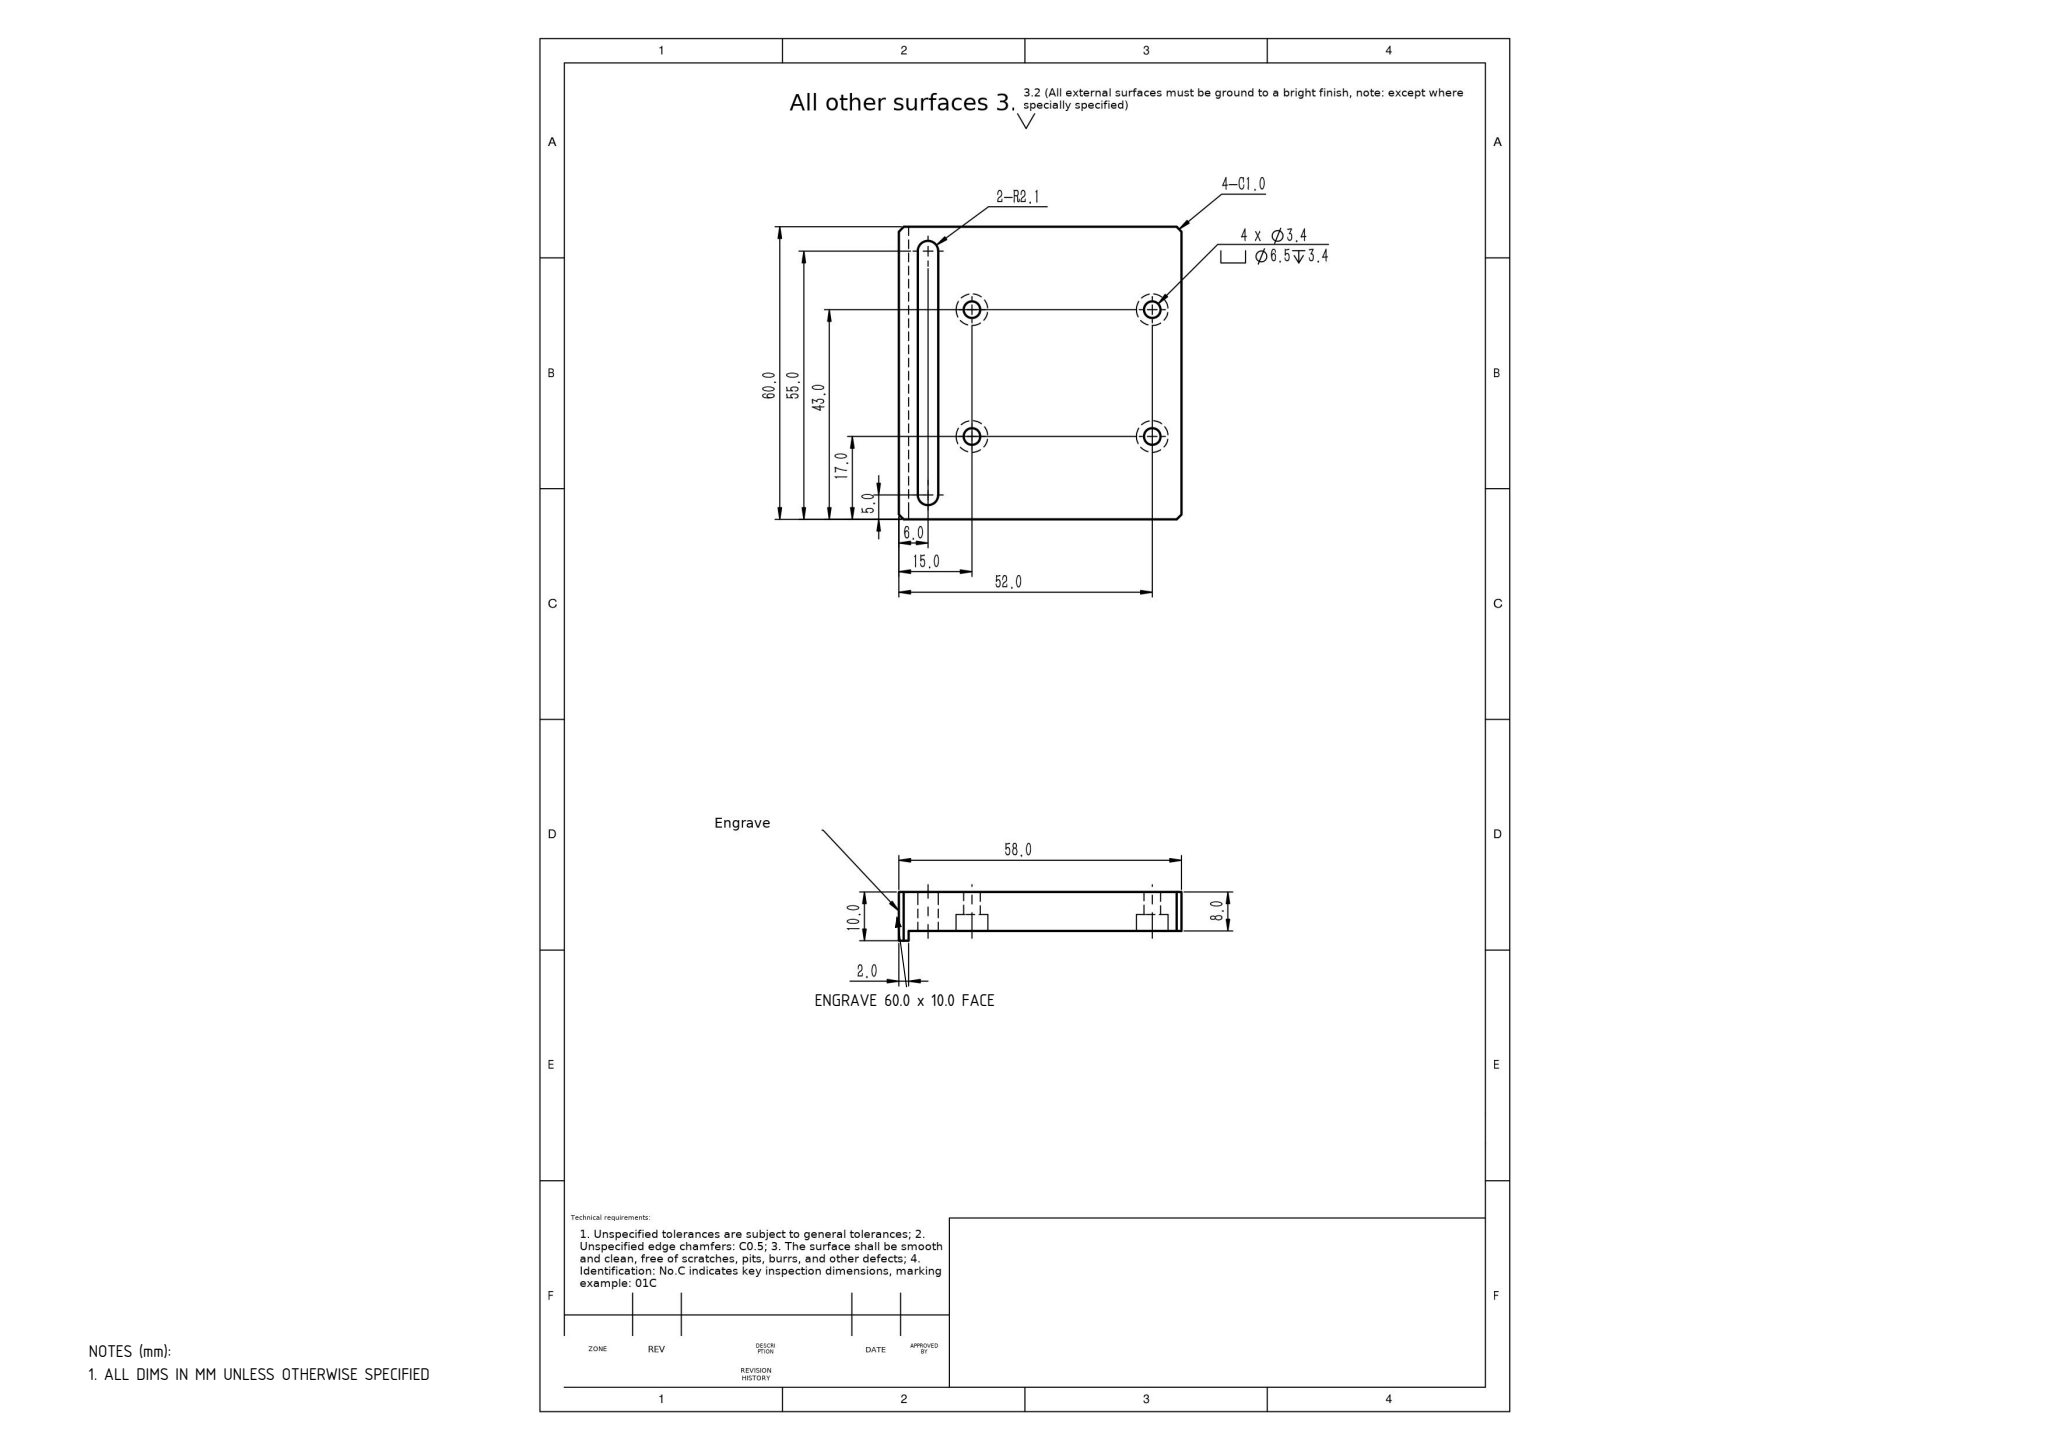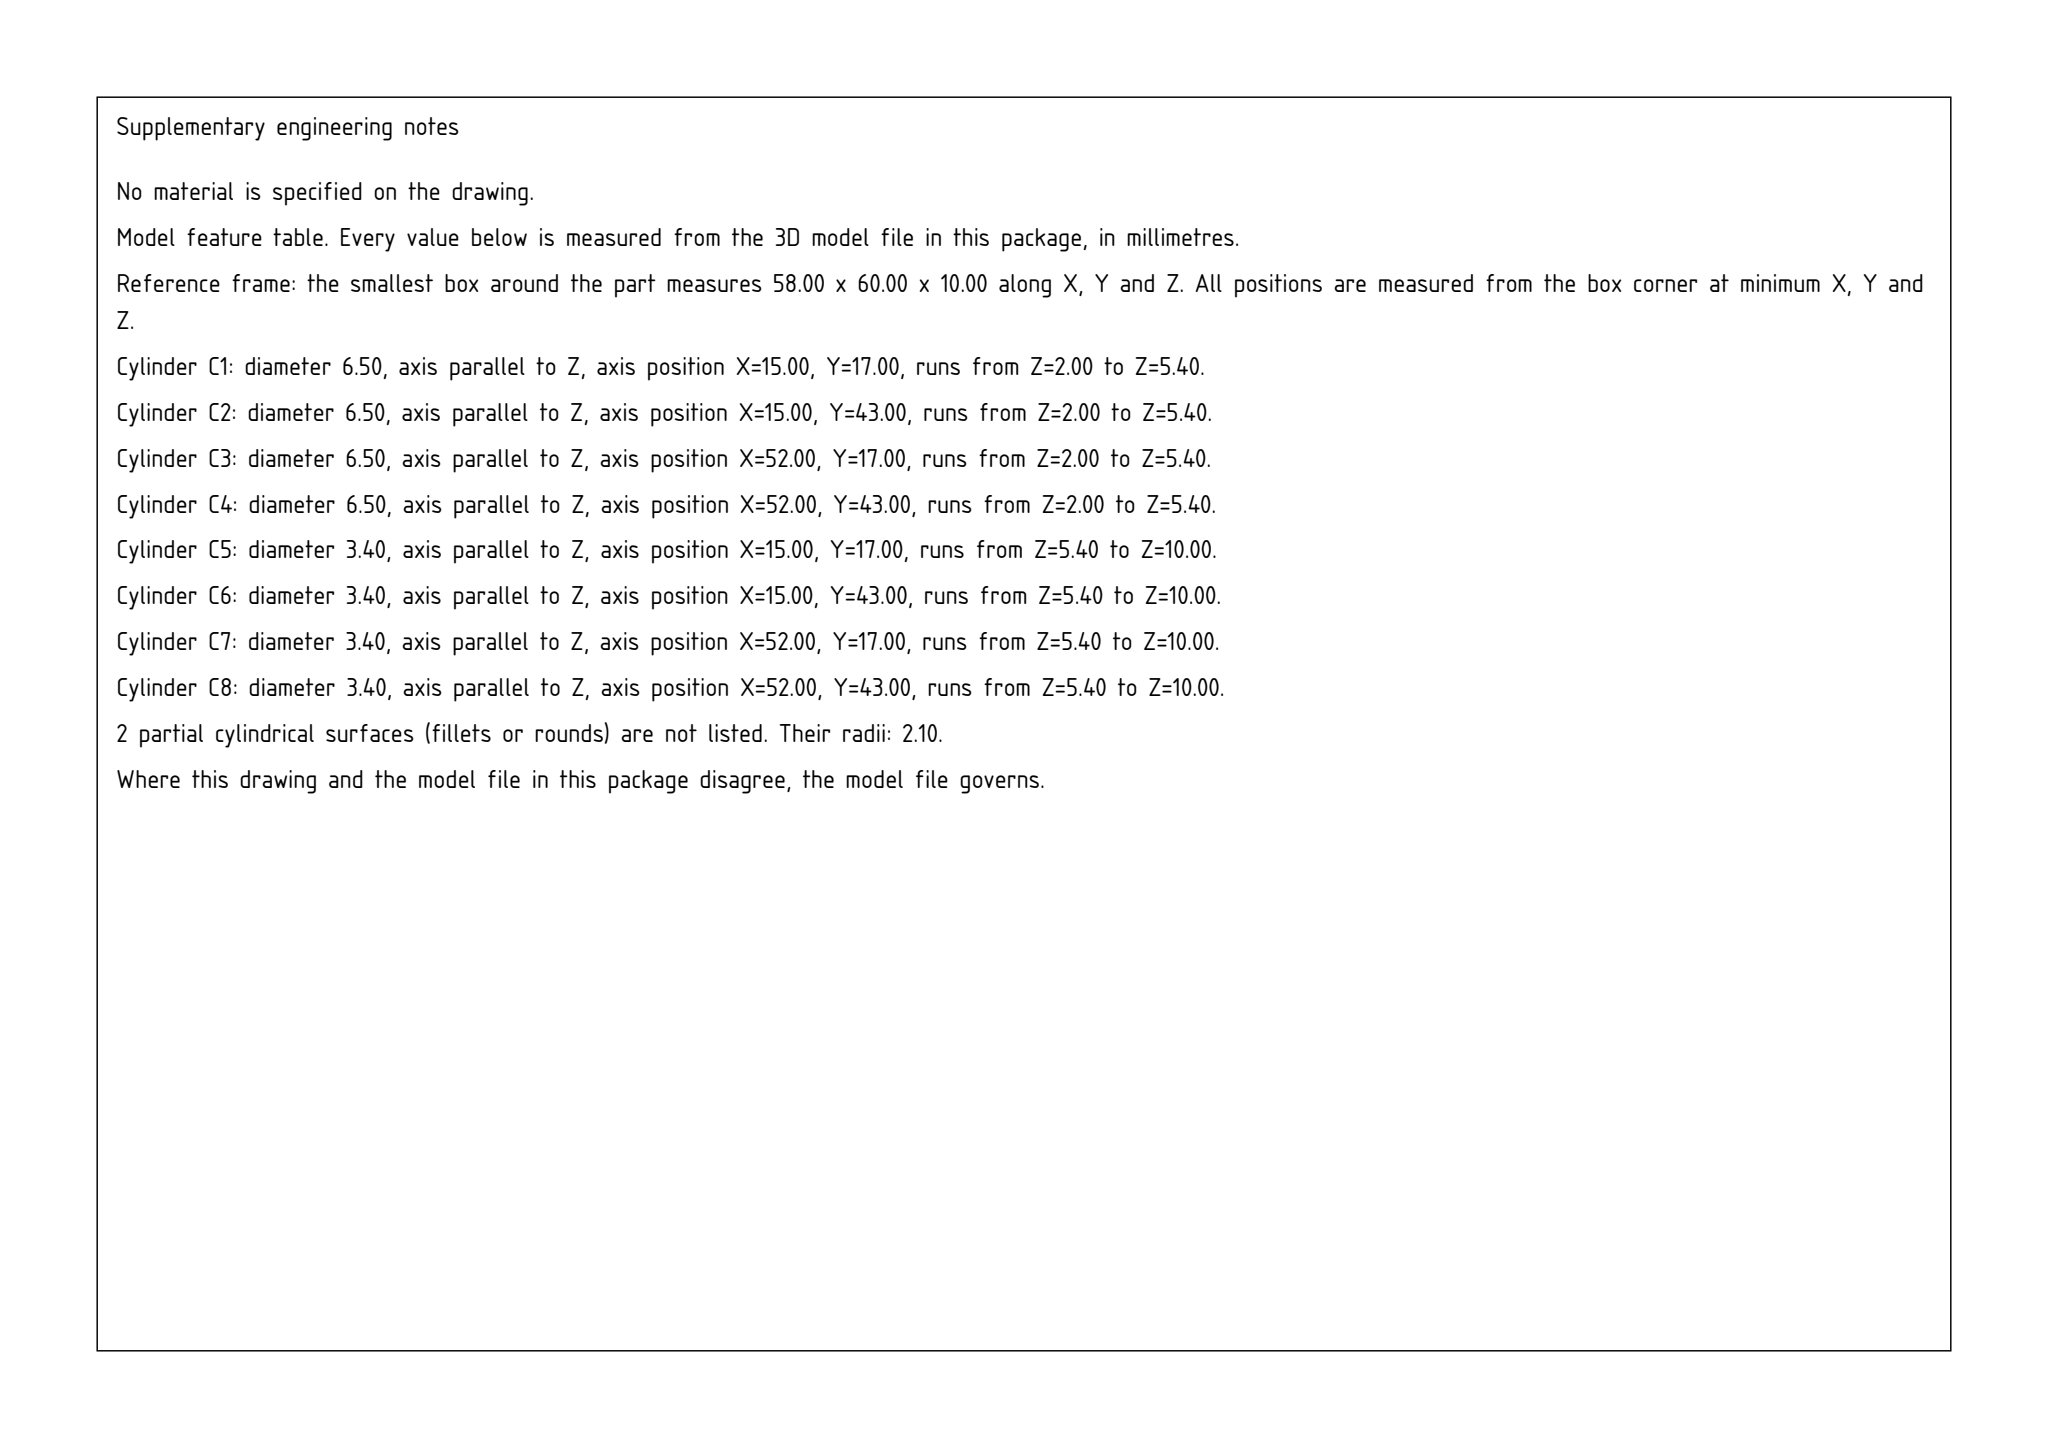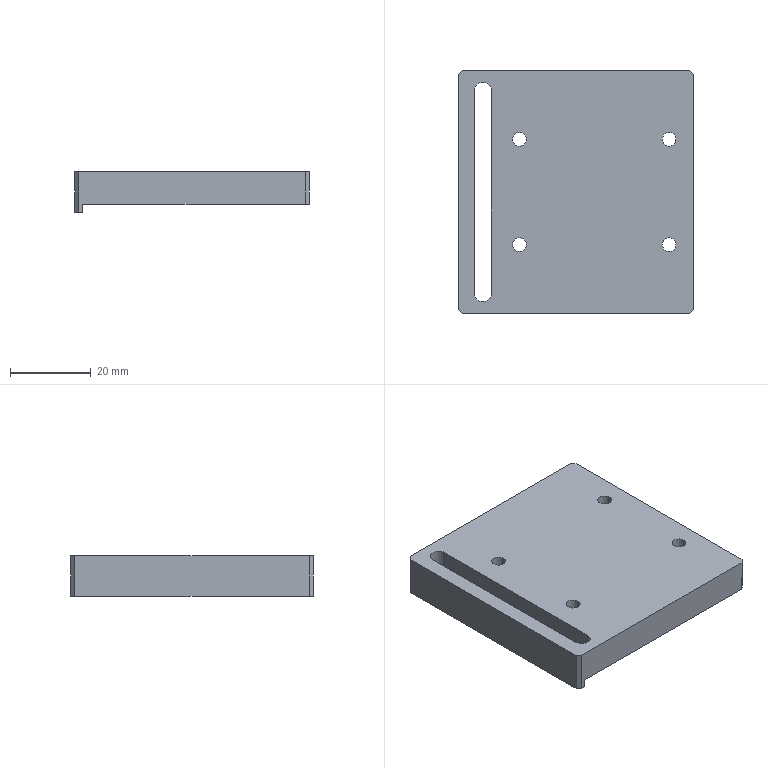Part | SolidWorks | mm | 1 solid | 36 faces | box 58 x 60 x 10 mm | volume 25653 mm3 | cylinder 18 | plane 18 | commonest cylinder face diameters 6.5 x8 3.4 x8 4.2 x2
Drawing notes:
ALL DIMS IN MM UNLESS OTHERWISE SPECIFIED | from the solid: STEP bbox 58.0 x 60.0 x 10.0 mm; all cyl dia 3.4/4.2/6.5 mm
ENGRAVE ON 2.0 THK LIP OUTER FACE, 60.0 x 10.0 AREA | from the solid: Plane normal x at offset 0.0, extent y[1,59] z[0,10]; lip thk 2.0 (plane z=2.0 starts at x=2.0)
build123d program:
from build123d import *

# Parameters (mm, degrees)
SKETCH1_W                                       = 58
SKETCH1_H                                       = 60
BOSS_EXTRUDE1_DEPTH                             = 8
SKETCH2_W                                       = 2
SKETCH2_H                                       = 60
BOSS_EXTRUDE2_DEPTH                             = 2
M3_HEX_SOCKET_HEAD_CAP_SCREW_CBORE1_D           = 3.4
M3_HEX_SOCKET_HEAD_CAP_SCREW_CBORE1_CBORE_D     = 6.5
M3_HEX_SOCKET_HEAD_CAP_SCREW_CBORE1_CBORE_DEPTH = 3.4
CUT_EXTRUDE4_DEPTH                              = 43.907
CHAMFER1_SIZE                                   = 1


with BuildPart() as part:
    # Sketch1 → Boss-Extrude1 (new body)
    with BuildSketch(Plane.XY):
        Rectangle(SKETCH1_W, SKETCH1_H)
    extrude(amount=BOSS_EXTRUDE1_DEPTH)

    # Sketch2 → Boss-Extrude2 (add)
    with BuildSketch(Plane(origin=(0, 0, 0), x_dir=(-1, 0, 0), z_dir=(0, 0, -1))):
        with Locations((28, 0)):
            Rectangle(SKETCH2_W, SKETCH2_H)
    extrude(amount=BOSS_EXTRUDE2_DEPTH)

    # M3 Hex Socket Head Cap Screw CBORE1 (through all)
    with Locations(Plane(origin=(0, 0, 0), x_dir=(-1, 0, 0), z_dir=(0, 0, -1))):
        with Locations((14, 13), (14, -13), (-23, -13), (-23, 13)):
            CounterBoreHole(M3_HEX_SOCKET_HEAD_CAP_SCREW_CBORE1_D / 2, M3_HEX_SOCKET_HEAD_CAP_SCREW_CBORE1_CBORE_D / 2, M3_HEX_SOCKET_HEAD_CAP_SCREW_CBORE1_CBORE_DEPTH)

    # Sketch5 → Cut-Extrude4 (cut, through all)
    with BuildSketch(Plane.XY.offset(8)):
        with BuildLine():
            Line((-20.9, 25), (-20.9, -25))
            ThreePointArc((-20.9, -25), (-23, -27.1), (-25.1, -25))
            Line((-25.1, -25), (-25.1, 25))
            ThreePointArc((-25.1, 25), (-23, 27.1), (-20.9, 25))
        make_face()
    extrude(amount=-CUT_EXTRUDE4_DEPTH, mode=Mode.SUBTRACT)

    # Chamfer1
    chamfer1_edges = [part.edges().sort_by_distance(p)[0] for p in [
        (-29, -30, 3),
        (-29, 30, 3),
        (29, -30, 4),
        (29, 30, 4),
    ]]
    chamfer(chamfer1_edges, length=CHAMFER1_SIZE)


solid = part.part